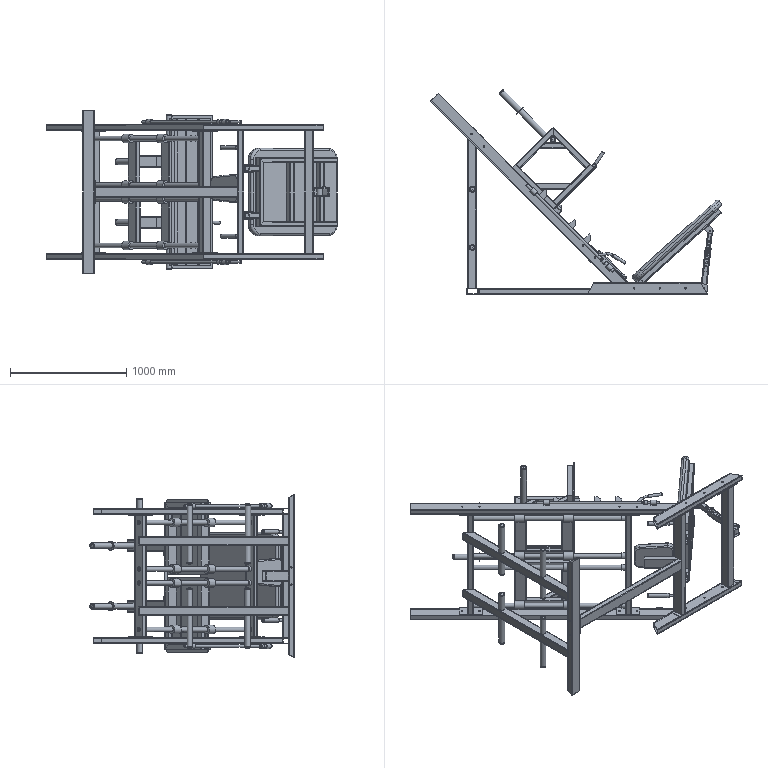Assembly | NX | mm | 118 component files | 118 solids | 1495 faces | box 2500.08 x 1756.4 x 1400 mm | volume 91637363 mm3 | plane 767 | cylinder 671 | spline 30 | torus 21 | cone 6 | commonest cylinder face diameters 8 x384 13 x80 50 x52 40 x24 42 x24 25 x21 20 x16 34 x14
Bill of materials:
unnamed part 1 | 4 |  | Short hollow cylinder (ring/sleeve) with a concentric through-bore and flat, square-cut end faces; length is roughly equal to or a little less than the outer diameter.
unnamed part 2 | 2 |  | Long straight square hollow tube with rounded outer and inner corners and square-cut ends.
unnamed part 3 | 2 |  | Headed cylindrical pin: a plain round shank with a thin, flat, larger-diameter disc head at one end; the far shank end looks lightly rounded or chamfered.
unnamed part 4 | 4 |  | Long straight rectangular (near-square) bar with slightly rounded longitudinal edges; each end face shows an inset rectangular border.
unnamed part 5 | 4 |  | Straight rectangular hollow tube with a thin wall, a section of about 2:1 aspect ratio, rounded corners and square-cut ends.
unnamed part 6 | 1 |  | Long rectangular hollow tube (rounded-rectangle section, about 2:1) with both ends cut at an angle in one plane and two small through-holes along one narrow face near mid-length.
unnamed part 7 | 1 |  | Thin, flat, roughly square plate with generously rounded corners and fully rounded or filleted perimeter edges.
unnamed part 8 | 2 |  | Solid plain cylinder (round rod segment) with flat end faces; length is roughly 2–3 times the diameter.
unnamed part 9 | 1 |  | Long straight rectangular hollow tube with a section of about 2:1, rounded corners, a moderate wall and square-cut ends.
unnamed part 10 | 4 |  | Square hollow tube with a thin wall and rounded corners; both ends are mitred in the same plane in opposite directions, giving a trapezoidal side profile.
unnamed part 11 | 2 |  | Thin, flat, nearly square plate with slightly rounded corners; three faint parallel lines run across each face.
unnamed part 12 | 1 |  | Long straight square hollow tube with rounded corners, a relatively thick wall and square-cut ends.
unnamed part 13 | 2 |  | Long, slender, straight member with a thin rectangular section and four small through holes on one wide face, set as two closely spaced pairs near each end; at least one end looks cut at an angle.
unnamed part 14 | 4 |  | Short length of hollow rectangular tube with rounded outer corners and both ends cut at an angle, so the side view is a trapezoid.
unnamed part 15 | 2 |  | Hollow rectangular tube with rounded corners, both ends cut at an angle (trapezoidal side view), and three evenly spaced through holes in a line on one wide face.
unnamed part 16 | 4 |  | Hollow rectangular tube with rounded corners. One end looks square-cut and the other angled in the isometric view.
unnamed part 17 | 2 |  | Straight round tube with a fairly thick wall and plain square-cut ends.
unnamed part 18 | 2 |  | U-shaped bent-plate bracket: two parallel legs joined by a flat web with inside bend radii. Each leg ends in a semicircular rounded tip with one through hole, and the two holes line up.
unnamed part 19 | 1 |  | Flat rectangular plate or bar with two round through holes on the longitudinal centerline, one near each end.
unnamed part 20 | 2 |  | Long, slender hollow rectangular tube with a small section, one end cut at an angle and the other end square-cut.
unnamed part 21 | 1 |  | U-shaped bent-plate bracket like a clevis-style form: two parallel legs on a flat web, each leg with a rounded end and one through hole. The legs look slightly tapered toward their rounded ends.
unnamed part 22 | 2 |  | Straight round tube with a relatively thin wall and plain square-cut ends.
unnamed part 23 | 2 |  | Short, thin-walled hollow rectangular section with rounded corners and both ends cut at an angle (trapezoidal side view).
unnamed part 24 | 2 |  | Flat rectangular plate with two round through holes on the longitudinal centerline, one near each short end.
unnamed part 25 | 2 |  | Long straight round rod or tube with four flat, evenly spaced tabs projecting from one side, a short collar near one end, and a bent round branch joining the main rod just above the collar to form a Y-shaped end.
unnamed part 26 | 1 |  | Length of square hollow tube with rounded corners and both ends cut at an angle (mitered).
unnamed part 27 | 2 |  | Length of rectangular/square hollow tube with rounded corners and both ends mitered in opposite directions, giving a trapezoidal side profile.
unnamed part 28 | 4 |  | Plain straight round tube with a small concentric bore, square-cut ends.
unnamed part 29 | 2 |  | Flat rectangular plate with two round through holes on the long centerline, one near each end.
unnamed part 30 | 1 |  | Rectangular block or thick pad with large corner radii and rounded edges all around.
unnamed part 31 | 2 |  | Long thin flat strip with three equally spaced round through holes on its centerline.
unnamed part 32 | 4 |  | Thick-walled cylindrical sleeve or bushing with a plain concentric bore and flat ends.
unnamed part 33 | 4 |  | Short thick-walled cylindrical spacer or tube with a concentric through bore and flat ends.
unnamed part 34 | 2 |  | Square hollow tube with rounded corners, two round holes through one face along its length, and one end cut at an angle.
unnamed part 35 | 1 |  | Rectangular hollow tube with rounded corners, one end cut at an angle and showing a V-shaped wall outline.
unnamed part 36 | 1 |  | Solid round rod bent into an L shape, with a long leg, a short leg and a tight bend of about 90 degrees.
unnamed part 37 | 2 |  | Straight, thin-walled round tube with plain square-cut open ends.
unnamed part 38 | 8 |  | Short, thick-walled cylindrical sleeve (a bushing- or spacer-like ring) with a central through bore.
unnamed part 39 | 1 |  | Square tube arm with rounded corners. A row of eight evenly spaced round holes runs along it, and a short round tubular collar is joined across one end with its axis perpendicular to the arm.
unnamed part 40 | 4 |  | Straight, thin-walled round tube with plain square-cut open ends.
unnamed part 41 | 14 |  | Shallow round disc or cap. One face has a recessed circular pocket inside a stepped rim, and the other face looks slightly domed or curved.
unnamed part 42 | 2 |  | Short length of rectangular or square tube with rounded corners and open ends, with a single round hole near one end.
unnamed part 43 | 1 |  | Straight bar with a rectangular section and rounded corners. It has a larger hollow cylindrical collar at one end and a small cylindrical boss with a small central hole on top near the other end.
unnamed part 44 | 2 |  | Straight round tube with open ends and a moderate wall thickness.
unnamed part 45 | 1 |  | U-shaped formed bracket (a channel or clevis-like shape). Two parallel D-shaped flanges with rounded ends are joined by a flat web with radiused bends, and each flange has a round hole; the two holes are aligned.
unnamed part 46 | 1 |  | Long, straight rectangular hollow tube with rounded corners, a thin wall and plain open ends.
unnamed part 47 | 1 |  | Straight rectangular hollow tube with rounded corners, a thin wall and plain open ends.
unnamed part 48 | 1 |  | Straight rectangular hollow tube with rounded corners and a thin wall, with four round holes spaced unevenly along its length.
Mates:
1. fix | vertical_bracket_base_beam 1 component
2. touch align | vertical_bracket_base_beam 1 | vertical_bracket_upright_beam 2
3. center | vertical_bracket_upright_beam 2 | vertical_bracket_upright_beam 2 | vertical_bracket_base_beam 1 | vertical_bracket_base_beam 1
4. touch align | vertical_bracket_base_beam 1 | vertical_bracket_upright_beam 1
5. center | vertical_bracket_upright_beam 1 | vertical_bracket_upright_beam 1 | vertical_bracket_base_beam 1 | vertical_bracket_base_beam 1
6. distance | vertical_bracket_upright_beam 2 | vertical_bracket_upright_beam 1
7. center | vertical_bracket_upright_beam 2 | vertical_bracket_upright_beam 1 | vertical_bracket_base_beam 1 | vertical_bracket_base_beam 1
8. center | vertical_bracket_conn_beam 1 | vertical_bracket_conn_beam 1 | vertical_bracket_upright_beam 1 | vertical_bracket_upright_beam 2
9. touch align | vertical_bracket_upright_beam 2 | vertical_bracket_conn_beam 1
10. distance | vertical_bracket_conn_beam 1 | vertical_bracket_upright_beam 2
11. touch align | conn_post 4 | vertical_bracket_upright_beam 2
12. distance | conn_post 4 | vertical_bracket_upright_beam 2
13. touch align | conn_post 3 | vertical_bracket_upright_beam 1
14. distance | conn_post 3 | vertical_bracket_upright_beam 1
15. touch align | conn_post 2 | vertical_bracket_upright_beam 2
16. touch align | conn_post 2 | conn_post 4
17. touch align | conn_post 1 | vertical_bracket_upright_beam 1
18. touch align | conn_post 1 | conn_post 3
19. touch align | vertical_bracket_conn_beam 1 | vertical_bracket_conn_plate 2
20. center | vertical_bracket_conn_beam 1 | vertical_bracket_conn_beam 1 | vertical_bracket_conn_plate 2 | vertical_bracket_conn_plate 2
21. touch align | vertical_bracket_conn_plate 2 | vertical_bracket_conn_beam 1
22. touch align | vertical_bracket_conn_plate 1 | vertical_bracket_conn_plate 2
23. touch align | vertical_bracket_conn_plate 1 | vertical_bracket_conn_plate 2
24. touch align | vertical_bracket_conn_plate 2 | vertical_bracket_conn_plate 1
25. fix | incl_supp_frame_bot_beam 1 component
26. touch align | incl_supp_frame_bot_beam 1 | incl_supp_frame_conn_beam 1
27. touch align | incl_supp_frame_conn_beam 1 | incl_supp_frame_bot_beam 1
28. distance | incl_supp_frame_conn_beam 1 | incl_supp_frame_bot_beam 1
29. touch align | incl_supp_frame_conn_col 2 | incl_supp_frame_conn_beam 1
30. touch align | incl_supp_frame_conn_col 2 | incl_supp_frame_conn_beam 1
31. distance | incl_supp_frame_conn_col 2 | incl_supp_frame_conn_beam 1
32. touch align | incl_supp_frame_conn_col 1 | incl_supp_frame_conn_col 2
33. distance | incl_supp_frame_conn_col 1 | incl_supp_frame_conn_col 2
34. fix | incl_supp_frame_bot_beam 1 component
35. touch align | incl_supp_frame_bot_beam 1 | incl_supp_frame_conn_beam 1
36. touch align | incl_supp_frame_conn_beam 1 | incl_supp_frame_bot_beam 1
37. distance | incl_supp_frame_conn_beam 1 | incl_supp_frame_bot_beam 1
38. touch align | incl_supp_frame_conn_col 2 | incl_supp_frame_conn_beam 1
39. touch align | incl_supp_frame_conn_col 2 | incl_supp_frame_conn_beam 1
40. distance | incl_supp_frame_conn_col 2 | incl_supp_frame_conn_beam 1
41. touch align | incl_supp_frame_conn_col 1 | incl_supp_frame_conn_col 2
42. distance | incl_supp_frame_conn_col 1 | incl_supp_frame_conn_col 2
43. fix | conn_frame_cross_beam 1 component
44. touch align | conn_frame_cross_beam 1 | conn_frame_conn_plate 2
45. touch align | conn_frame_conn_plate 2 | conn_frame_cross_beam 1
46. center | conn_frame_conn_plate 2 | conn_frame_conn_plate 2 | conn_frame_cross_beam 1 | conn_frame_cross_beam 1
47. touch align | conn_frame_conn_plate 1 | conn_frame_cross_beam 1
48. touch align | conn_frame_conn_plate 1 | conn_frame_cross_beam 1
49. center | conn_frame_conn_plate 1 | conn_frame_conn_plate 1 | conn_frame_cross_beam 1 | conn_frame_cross_beam 1
50. touch align | conn_frame_cross_beam 1 | conn_frame_conn_post 4
51. distance | conn_frame_conn_post 4 | conn_frame_cross_beam 1
52. distance | conn_frame_conn_post 4 | conn_frame_conn_plate 2
53. touch align | conn_frame_cross_beam 1 | conn_frame_conn_post 3
54. distance | conn_frame_conn_post 3 | conn_frame_cross_beam 1
55. distance | conn_frame_conn_post 3 | conn_frame_conn_post 4
56. touch align | conn_frame_cross_beam 1 | conn_frame_conn_post 2
57. distance | conn_frame_conn_post 2 | conn_frame_cross_beam 1
58. distance | conn_frame_conn_post 3 | conn_frame_conn_post 2
59. touch align | conn_frame_cross_beam 1 | conn_frame_conn_post 1
60. distance | conn_frame_conn_post 1 | conn_frame_cross_beam 1
61. distance | conn_frame_conn_post 2 | conn_frame_conn_post 1
62. fix | adj_brkt_bot_beam 1 component
63. touch align | adj_brkt_bot_beam 1 | adj_brkt_vert_beam 2
64. touch align | adj_brkt_vert_beam 2 | adj_brkt_bot_beam 1
65. touch align | adj_brkt_vert_beam 2 | adj_brkt_bot_beam 1
66. touch align | adj_brkt_bot_beam 1 | adj_brkt_vert_beam 1
67. touch align | adj_brkt_vert_beam 1 | adj_brkt_bot_beam 1
68. touch align | adj_brkt_bot_beam 1 | adj_brkt_vert_beam 1
69. touch align | adj_brkt_vert_beam 1 | adj_brkt_top_beam 2
70. touch align | adj_brkt_top_beam 2 | adj_brkt_vert_beam 1
71. distance | adj_brkt_top_beam 2 | adj_brkt_vert_beam 1
72. touch align | adj_brkt_top_beam 1 | adj_brkt_vert_beam 2
73. touch align | adj_brkt_top_beam 1 | adj_brkt_top_beam 2
74. distance | adj_brkt_top_beam 2 | adj_brkt_top_beam 1
75. touch align | adj_brkt_top_beam 2 | adj_brkt_conn_lug 1
76. touch align | adj_brkt_conn_lug 1 | adj_brkt_top_beam 2
77. center | adj_brkt_conn_lug 1 | adj_brkt_conn_lug 1 | adj_brkt_vert_beam 1 | adj_brkt_vert_beam 2
78. touch align | adj_brkt_conn_beam 2 | adj_brkt_bot_beam 1
79. touch align | adj_brkt_conn_beam 2 | adj_brkt_bot_beam 1
80. touch align | adj_brkt_conn_beam 1 | adj_brkt_bot_beam 1
81. touch align | adj_brkt_conn_beam 1 | adj_brkt_conn_beam 2
82. distance | adj_brkt_conn_beam 1 | adj_brkt_conn_beam 2
83. center | adj_brkt_conn_beam 2 | adj_brkt_conn_beam 1 | adj_brkt_vert_beam 1 | adj_brkt_vert_beam 2
84. fix | slid_frame_bot_beam 2 component
85. touch align | slider_frame_conn_beam 2 | slid_frame_bot_beam 2
86. touch align | slider_frame_conn_beam 2 | slid_frame_bot_beam 2
87. touch align | slider_frame_conn_beam 2 | slid_frame_bot_beam 2
88. touch align | slid_frame_bot_beam 1 | slider_frame_conn_beam 2
89. touch align | slid_frame_bot_beam 1 | slider_frame_conn_beam 2
90. touch align | slid_frame_bot_beam 1 | slider_frame_conn_beam 2
91. touch align | slider_frame_conn_beam 1 | slid_frame_bot_beam 1
92. touch align | slider_frame_conn_beam 1 | slid_frame_bot_beam 1
93. touch align | slider_frame_conn_beam 1 | slid_frame_bot_beam 2
94. touch align | slid_frame_slid_ring 4 | slid_frame_bot_beam 2
95. touch align | slid_frame_slid_ring 4 | slid_frame_bot_beam 2
96. touch align | slid_frame_slid_ring 3 | slid_frame_bot_beam 2
97. touch align | slid_frame_slid_ring 3 | slid_frame_bot_beam 2
98. touch align | slid_frame_slid_ring 2 | slid_frame_bot_beam 1
99. touch align | slid_frame_slid_ring 2 | slid_frame_slid_ring 4
100. touch align | slid_frame_slid_ring 1 | slid_frame_bot_beam 1
101. touch align | slid_frame_slid_ring 1 | slid_frame_bot_beam 1
102. touch align | slid_frame_beam1 2 | slider_frame_conn_beam 2
103. touch align | slid_frame_beam1 2 | slider_frame_conn_beam 2
104. touch align | slid_frame_beam1 2 | slid_frame_bot_beam 2
105. touch align | slider_frame_conn_beam 1 | slid_frame_beam2 2
106. touch align | slid_frame_beam2 2 | slider_frame_conn_beam 1
107. center | slid_frame_beam2 2 | slid_frame_beam2 2 | slid_frame_bot_beam 2 | slid_frame_bot_beam 1
108. touch align | slid_frame_beam2 1 | slid_frame_beam2 2
109. touch align | slid_frame_beam2 1 | slid_frame_beam2 2
110. touch align | slid_frame_beam2 1 | slid_frame_beam2 2
111. touch align | slid_frame_beam3 1 | slid_frame_beam2 1
112. touch align | slid_frame_beam3 1 | slid_frame_beam2 1
113. touch align | slid_frame_beam3 1 | slid_frame_beam2 2
114. touch align | slid_frame_beam4 2 | slid_frame_beam1 2
115. touch align | slid_frame_beam4 2 | slid_frame_beam1 2
116. touch align | slid_frame_beam4 2 | slid_frame_beam1 2
117. touch align | slid_frame_beam4 1 | slid_frame_beam1 2
118. touch align | slid_frame_beam4 1 | slid_frame_beam1 2
119. touch align | slid_frame_beam1 2 | slid_frame_beam4 1
120. touch align | slid_frame_beam1 1 | slid_frame_beam4 2
121. touch align | slid_frame_beam1 1 | slid_frame_beam4 2
122. touch align | slid_frame_beam1 1 | slid_frame_beam4 2
123. touch align | pedal 1 | slid_frame_beam1 1
124. center | pedal 1 | pedal 1 | slid_frame_beam4 1 | slid_frame_beam4 2
125. center | pedal 1 | pedal 1 | slid_frame_beam1 2 | slid_frame_beam1 1
126. touch align | slid_frame_conn_col 1 | slid_frame_beam3 1
127. touch align | slid_frame_conn_col 1 | slid_frame_beam2 2
128. distance | slid_frame_conn_col 1 | slid_frame_beam2 1
129. touch align | slid_frame_beam5 1 | slid_frame_bot_beam 1
130. touch align | slid_frame_beam5 1 | slid_frame_bot_beam 1
131. touch align | pedal 1 | slid_frame_beam5 1
132. touch align | slid_frame_beam2 2 | slid_frame_conn_col2 1
133. distance | slid_frame_conn_col2 1 | slid_frame_beam2 1
134. distance | slid_frame_conn_col2 1 | slid_frame_beam2 2
135. concentric | slid_frame_supp_col 1 | slid_frame_conn_col2 1
136. touch align | pedal 1 | slider_frame_pin 1
137. distance | slider_frame_pin 1 | pedal 1
138. distance | slider_frame_pin 1 | pedal 1
139. touch align | slider_frame_conn_ring 2 | slid_frame_beam1 1
140. touch align | slider_frame_conn_ring 2 | pedal 1
141. touch align | slider_frame_conn_ring 2 | slid_frame_beam4 1
142. touch align | slider_frame_conn_ring 1 | slider_frame_conn_ring 2
143. distance | slider_frame_conn_ring 1 | slider_frame_conn_ring 2
144. distance | slid_frame_slid_ring 4 | slid_frame_bot_beam 2
145. distance | slid_frame_slid_ring 2 | slid_frame_bot_beam 1
146. touch align | slid_frame_slid_ring 3 | slid_frame_slid_ring 4
147. touch align | slid_frame_slid_ring 1 | slid_frame_slid_ring 2
148. fix | slid_frame_bot_beam 2 component
149. touch align | slider_frame_conn_beam 2 | slid_frame_bot_beam 2
150. touch align | slider_frame_conn_beam 2 | slid_frame_bot_beam 2
151. touch align | slider_frame_conn_beam 2 | slid_frame_bot_beam 2
152. touch align | slid_frame_bot_beam 1 | slider_frame_conn_beam 2
153. touch align | slid_frame_bot_beam 1 | slider_frame_conn_beam 2
154. touch align | slid_frame_bot_beam 1 | slider_frame_conn_beam 2
155. touch align | slider_frame_conn_beam 1 | slid_frame_bot_beam 1
156. touch align | slider_frame_conn_beam 1 | slid_frame_bot_beam 1
157. touch align | slider_frame_conn_beam 1 | slid_frame_bot_beam 2
158. touch align | slid_frame_slid_ring 4 | slid_frame_bot_beam 2
159. touch align | slid_frame_slid_ring 4 | slid_frame_bot_beam 2
160. touch align | slid_frame_slid_ring 3 | slid_frame_bot_beam 2
161. touch align | slid_frame_slid_ring 3 | slid_frame_bot_beam 2
162. touch align | slid_frame_slid_ring 2 | slid_frame_bot_beam 1
163. touch align | slid_frame_slid_ring 2 | slid_frame_slid_ring 4
164. touch align | slid_frame_slid_ring 1 | slid_frame_bot_beam 1
165. touch align | slid_frame_slid_ring 1 | slid_frame_bot_beam 1
166. touch align | slider_frame_conn_beam 1 | slid_frame_beam2 2
167. touch align | slid_frame_beam2 2 | slider_frame_conn_beam 1
168. center | slid_frame_beam2 2 | slid_frame_beam2 2 | slid_frame_bot_beam 2 | slid_frame_bot_beam 1
169. touch align | slid_frame_beam2 1 | slid_frame_beam2 2
170. touch align | slid_frame_beam2 1 | slid_frame_beam2 2
171. touch align | slid_frame_beam2 1 | slid_frame_beam2 2
172. touch align | slid_frame_beam3 1 | slid_frame_beam2 1
173. touch align | slid_frame_beam3 1 | slid_frame_beam2 1
174. touch align | slid_frame_beam3 1 | slid_frame_beam2 2
175. touch align | slid_frame_conn_col 1 | slid_frame_beam3 1
176. touch align | slid_frame_conn_col 1 | slid_frame_beam2 2
177. touch align | slid_frame_beam2 2 | slid_frame_conn_col2 1
178. distance | slid_frame_conn_col2 1 | slid_frame_beam2 1
179. distance | slid_frame_conn_col2 1 | slid_frame_beam2 2
180. concentric | slid_frame_supp_col 1 | slid_frame_conn_col2 1
181. distance | slid_frame_slid_ring 4 | slid_frame_bot_beam 2
182. distance | slid_frame_slid_ring 2 | slid_frame_bot_beam 1
183. touch align | slid_frame_slid_ring 3 | slid_frame_slid_ring 4
184. touch align | slid_frame_slid_ring 1 | slid_frame_slid_ring 2
185. distance | slid_frame_conn_col 1 | slid_frame_beam2 1
186. touch align | slider_frame_conn_beam 2 | slid_frame_beam1 2
187. touch align | slid_frame_beam1 2 | slider_frame_conn_beam 2
188. touch align | slid_frame_bot_beam 1 | slid_frame_beam1 2
189. touch align | slid_frame_beam1 2 | slid_frame_beam4 2
190. touch align | slid_frame_beam4 2 | slid_frame_beam1 2
191. touch align | slid_frame_beam4 2 | slid_frame_beam1 2
192. touch align | slid_frame_beam4 1 | slid_frame_beam1 2
193. touch align | slid_frame_beam4 1 | slid_frame_beam1 2
194. touch align | slid_frame_beam1 1 | slid_frame_beam4 2
195. touch align | slid_frame_beam1 1 | slid_frame_beam4 2
196. touch align | slid_frame_beam1 1 | slid_frame_beam4 2
197. touch align | slid_frame_beam4 1 | slid_frame_beam1 2
198. touch align | slid_frame_beam1 1 | pedal 1
199. center | pedal 1 | pedal 1 | slid_frame_beam4 1 | slid_frame_beam4 2
200. center | pedal 1 | pedal 1 | slid_frame_beam1 2 | slid_frame_beam1 1
201. touch align | pedal 1 | slider_frame_pin 1
202. distance | slider_frame_pin 1 | pedal 1
203. distance | slider_frame_pin 1 | pedal 1
204. touch align | slider_frame_conn_ring 2 | slid_frame_beam1 1
205. touch align | slider_frame_conn_ring 2 | pedal 1
206. touch align | slider_frame_conn_ring 1 | slider_frame_conn_ring 2
207. distance | slider_frame_conn_ring 1 | slider_frame_conn_ring 2
208. touch align | slider_frame_conn_ring 1 | slid_frame_beam4 1
209. touch align | slid_frame_bot_beam 2 | slid_frame_beam5 1
210. touch align | slid_frame_beam5 1 | slid_frame_bot_beam 2
211. touch align | pedal 1 | slid_frame_beam5 1
212. fix | base_frame_rect_tube 1 component
213. parallel | base_frame_sq_tube 1 face | base_frame_rect_tube 1 face
214. center | base_frame_sq_tube 1 face | base_frame_sq_tube 1 face | base_frame_rect_tube 1 face | base_frame_rect_tube 1 face
215. center | base_frame_sq_tube 1 face | base_frame_sq_tube 1 face | base_frame_rect_tube 1 face | base_frame_rect_tube 1 face
216. touch align | base_frame_rect_tube 1 face | side_conn_plate 2 face
217. center | side_conn_plate 2 face | side_conn_plate 2 face | base_frame_rect_tube 1 face | base_frame_rect_tube 1 face
218. center | side_conn_plate 2 face | side_conn_plate 2 face | base_frame_rect_tube 1 face | base_frame_sq_tube 1 face
219. distance | base_frame_rect_tube 1 face | base_frame_sq_tube 1 face
220. touch align | side_conn_plate 1 face | base_frame_sq_tube 1 face
221. touch align | side_conn_plate 1 face | side_conn_plate 2 face
222. touch align | side_conn_plate 1 face | side_conn_plate 2 face
223. touch align | base_frame_rect_tube2 1 face | base_frame_rect_tube 1 face
224. center | base_frame_rect_tube2 1 face | base_frame_rect_tube2 1 face | side_conn_plate 2 face | side_conn_plate 1 face
225. touch align | base_frame_rect_tube 1 face | base_frame_rect_tube2 1 face
226. touch align | base_frame_short_conn_plate 1 face | base_frame_rect_tube2 1 face
227. center | base_frame_short_conn_plate 1 face | base_frame_short_conn_plate 1 face | base_frame_rect_tube2 1 face | base_frame_rect_tube2 1 face
228. center | base_frame_short_conn_plate 1 face | base_frame_short_conn_plate 1 face | base_frame_rect_tube2 1 face | base_frame_rect_tube2 1 face
229. touch align | base_frame_rect_tube 1 face | base_frame_rnd_tube 2 face
230. parallel | base_frame_rnd_tube 2 datumplane | side_conn_plate 1 face
231. touch align | base_frame_rect_tube 1 face | base_frame_rnd_tube 1 face
232. parallel | base_frame_rnd_tube 1 datumplane | side_conn_plate 2 face
233. distance | base_frame_rnd_tube 2 face | base_frame_rnd_tube 1 face
234. center | base_frame_rnd_tube 1 face | base_frame_rnd_tube 2 face | side_conn_plate 1 face | side_conn_plate 2 face
235. touch align | base_frame_rnd_tube 1 face | base_frame_rect_tube 1 edge
236. touch align | base_frame_rnd_tube 1 datumplane | base_frame_rnd_tube 2 datumplane
237. center | base_frame_rect_tube3 1 face | base_frame_rect_tube3 1 face | base_frame_rect_tube2 1 face | base_frame_rect_tube2 1 face
238. touch align | base_frame_rect_tube2 1 face | base_frame_rect_tube3 1 face
239. touch align | base_frame_rect_tube3 1 face | base_frame_rect_tube 1 face
240. touch align | base_frame_sq_tube 1 face | base_frame_conn 1 face
241. center | base_frame_conn 1 face | base_frame_conn 1 face | base_frame_sq_tube 1 face | base_frame_sq_tube 1 face
242. center | base_frame_conn 1 face | base_frame_conn 1 face | side_conn_plate 2 face | side_conn_plate 1 face
243. touch align | base_frame_rect_tube 1 face | base_frame_conn2 2 face
244. center | base_frame_conn2 2 face | base_frame_conn2 2 face | base_frame_rect_tube 1 face | base_frame_rect_tube 1 face
245. touch align | base_frame_rect_tube 1 face | base_frame_conn2 1 face
246. center | base_frame_conn2 1 face | base_frame_conn2 1 face | base_frame_rect_tube 1 face | base_frame_rect_tube 1 face
247. distance | base_frame_conn2 2 face | base_frame_conn2 1 edge
248. center | base_frame_conn2 1 face | base_frame_conn2 2 face | side_conn_plate 1 face | side_conn_plate 2 face
249. concentric | vertical_bracket_assy 1 arc | base_frame_short_conn_plate 1 edge
250. parallel | vertical_bracket_assy 1 face | base_frame_rect_tube2 1 face
251. concentric | incl_supp_frame_assy 1 edge | side_conn_plate 2 edge
252. parallel | incl_supp_frame_assy 1 face | base_frame_rect_tube 1 face
253. concentric | incl_supp_frame_assy2 1 arc | side_conn_plate 1 edge
254. parallel | incl_supp_frame_assy2 1 face | base_frame_rect_tube 1 face
255. concentric | conn_frame_assy 1 edge | incl_supp_frame_assy 1 edge
256. parallel | conn_frame_assy 1 face | incl_supp_frame_assy 1 face
257. touch align | adj_brkt_assy 1 face | base_frame_conn2 1 face
258. center | adj_brkt_assy 1 face | adj_brkt_assy 1 face | base_frame_conn2 2 face | base_frame_conn2 1 face
259. touch align | lying_cushion 1 face | adj_brkt_assy 1 face
260. center | lying_cushion 1 face | lying_cushion 1 face | adj_brkt_assy 1 face | adj_brkt_assy 1 face
261. distance | lying_cushion 1 face | adj_brkt_assy 1 face
262. touch align | adj_rod_out_frame 1 face | base_frame_conn 1 face
263. center | adj_rod_out_frame 1 face | adj_rod_out_frame 1 face | base_frame_conn 1 face | base_frame_conn 1 face
264. center | adj_inner_brkt 1 face | adj_inner_brkt 1 face | adj_rod_out_frame 1 face | adj_rod_out_frame 1 face
265. center | adj_inner_brkt 1 face | adj_inner_brkt 1 face | adj_rod_out_frame 1 face | adj_rod_out_frame 1 face
266. touch align | adj_inner_brkt 1 face | adj_brkt_assy 1 face
267. concentric | sliding_post 4 edge | conn_frame_assy 1 edge
268. concentric | sliding_post 3 edge | conn_frame_assy 1 edge
269. concentric | sliding_post 2 edge | conn_frame_assy 1 edge
270. concentric | sliding_post 1 edge | conn_frame_assy 1 edge
271. touch align | seat_cush 1 face | base_frame_rect_tube3 1 face
272. touch align | seat_cush 1 face | base_frame_rect_tube 1 face
273. center | seat_cush 1 face | seat_cush 1 face | incl_supp_frame_assy 1 face | incl_supp_frame_assy2 1 face
274. touch align | slid_frame_assy 1 face | sliding_post 3 face
275. parallel | slid_frame_assy 1 face | incl_supp_frame_assy2 1 face
276. touch align | slid_frame_assy2 1 face | sliding_post 2 face
277. parallel | slid_frame_assy2 1 face | incl_supp_frame_assy 1 face
278. touch align | slid_frame_assy2 1 face | slid_frame_assy 1 face
279. touch align | pin 1 face | slid_frame_assy2 1 face
280. touch align | pos_push_rod 2 face | incl_supp_frame_assy 1 face
281. parallel | pos_push_rod 2 face | incl_supp_frame_assy 1 face
282. touch align | slid_frame_assy2 1 face | pos_push_rod 2 face
283. distance | pos_push_rod 2 face | incl_supp_frame_assy 1 face
284. touch align | pos_push_rod 1 face | incl_supp_frame_assy2 1 face
285. parallel | pos_push_rod 1 face | incl_supp_frame_assy2 1 face
286. touch align | slid_frame_assy 1 face | pos_push_rod 1 face
287. concentric | end_cap 14 edge | vertical_bracket_assy 1 edge
288. concentric | end_cap 13 edge | vertical_bracket_assy 1 edge
289. concentric | end_cap 12 edge | vertical_bracket_assy 1 edge
290. concentric | end_cap 11 edge | vertical_bracket_assy 1 edge
291. concentric | end_cap 10 edge | vertical_bracket_assy 1 edge
292. concentric | end_cap 9 edge | vertical_bracket_assy 1 edge
293. concentric | end_cap 8 edge | vertical_bracket_assy 1 edge
294. concentric | end_cap 7 edge | vertical_bracket_assy 1 edge
295. concentric | end_cap 6 edge | slid_frame_assy 1 edge
296. concentric | end_cap 5 edge | slid_frame_assy 1 edge
297. concentric | slid_frame_assy2 1 edge | end_cap 4 edge
298. concentric | end_cap 3 edge | slid_frame_assy2 1 edge
299. concentric | end_cap 2 edge | slid_frame_assy 1 edge
300. concentric | end_cap 1 edge | slid_frame_assy2 1 edge
301. concentric | grip 2 edge | base_frame_rnd_tube 1 edge
302. concentric | grip 1 edge | base_frame_rnd_tube 2 edge